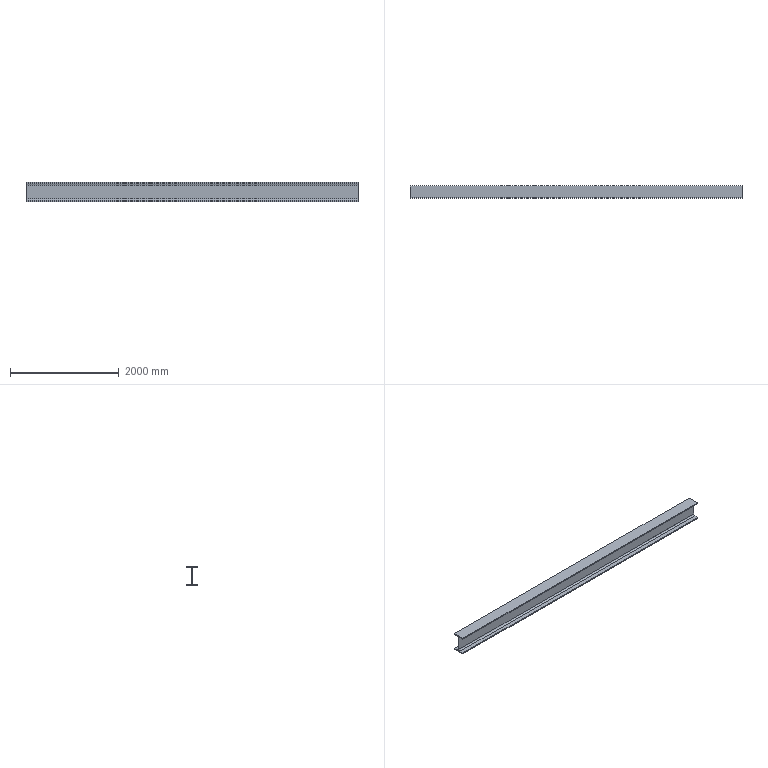Component | SolidWorks | OriginalColumn-2 | 1 solid | 18 faces | box 6100 x 220 x 350 mm | volume 80477247 mm3 | plane 14 | cylinder 4 | commonest cylinder face diameters 56 x4
build123d program:
from build123d import *

# Parameters (mm, degrees)
H_BEAM_HM600_300B_1_DEPTH = 6100


with BuildPart() as part:
    # Sketch1 → H-Beam HM600_300B_1 (new body)
    with BuildSketch(Plane.YZ):
        with BuildLine():
            Line((-110, -175), (-110, -155))
            Line((-110, -155), (-34, -155))
            ThreePointArc((-34, -155), (-14.201, -146.799), (-6, -127))
            Line((-6, -127), (-6, 127))
            ThreePointArc((-6, 127), (-14.201, 146.799), (-34, 155))
            Line((-34, 155), (-110, 155))
            Line((-110, 155), (-110, 175))
            Line((-110, 175), (110, 175))
            Line((110, 175), (110, 155))
            Line((110, 155), (34, 155))
            ThreePointArc((34, 155), (14.201, 146.799), (6, 127))
            Line((6, 127), (6, -127))
            ThreePointArc((6, -127), (14.201, -146.799), (34, -155))
            Line((34, -155), (110, -155))
            Line((110, -155), (110, -175))
            Line((110, -175), (-110, -175))
        make_face()
    extrude(amount=H_BEAM_HM600_300B_1_DEPTH)


solid = part.part

# Placed as in the assembly
solid = solid.moved(Location((-1730.074, -5132.346, -322.679), (0, 0, 0)))
STEP:
#1=COLOUR_RGB('',0.7922,0.8196,0.9333);
#2=FILL_AREA_STYLE_COLOUR('',#1);
#3=FILL_AREA_STYLE('',(#2));
#4=SURFACE_STYLE_FILL_AREA(#3);
#5=SURFACE_SIDE_STYLE('',(#4));
#6=SURFACE_STYLE_USAGE(.BOTH.,#5);
#7=PRESENTATION_STYLE_ASSIGNMENT((#6));
#8=CARTESIAN_POINT('',(-68.113,-206.392,-19.594));
#9=VERTEX_POINT('',#8);
#10=CARTESIAN_POINT('',(-68.113,-197.73,-19.594));
#11=VERTEX_POINT('',#10);
#12=CARTESIAN_POINT('',(-68.113,-197.73,-19.594));
#13=DIRECTION('',(0.,1.,0.));
#14=VECTOR('',#13,39.37);
#15=LINE('',#12,#14);
#16=EDGE_CURVE('',#9,#11,#15,.T.);
#17=ORIENTED_EDGE('',*,*,#16,.T.);
#18=CARTESIAN_POINT('',(172.044,-197.73,-19.594));
#19=VERTEX_POINT('',#18);
#20=CARTESIAN_POINT('',(172.044,-197.73,-19.594));
#21=DIRECTION('',(-1.,0.,0.));
#22=VECTOR('',#21,39.37);
#23=LINE('',#20,#22);
#24=EDGE_CURVE('',#19,#11,#23,.T.);
#25=ORIENTED_EDGE('',*,*,#24,.F.);
#26=CARTESIAN_POINT('',(172.044,-206.392,-19.594));
#27=VERTEX_POINT('',#26);
#28=CARTESIAN_POINT('',(172.044,-197.73,-19.594));
#29=DIRECTION('',(0.,1.,0.));
#30=VECTOR('',#29,39.37);
#31=LINE('',#28,#30);
#32=EDGE_CURVE('',#27,#19,#31,.T.);
#33=ORIENTED_EDGE('',*,*,#32,.F.);
#34=CARTESIAN_POINT('',(172.044,-206.392,-19.594));
#35=DIRECTION('',(-1.,0.,0.));
#36=VECTOR('',#35,39.37);
#37=LINE('',#34,#36);
#38=EDGE_CURVE('',#27,#9,#37,.T.);
#39=ORIENTED_EDGE('',*,*,#38,.T.);
#40=EDGE_LOOP('',(#17,#25,#33,#39));
#41=FACE_OUTER_BOUND('',#40,.T.);
#42=CARTESIAN_POINT('',(172.044,-197.73,-19.594));
#43=DIRECTION('',(0.,0.,1.));
#44=DIRECTION('',(1.,0.,0.));
#45=AXIS2_PLACEMENT_3D('',#42,#43,#44);
#46=PLANE('',#45);
#47=ADVANCED_FACE('',(#41),#46,.F.);
#48=CARTESIAN_POINT('',(-68.113,-197.73,-18.806));
#49=VERTEX_POINT('',#48);
#50=CARTESIAN_POINT('',(-68.113,-197.73,-18.806));
#51=DIRECTION('',(0.,0.,1.));
#52=VECTOR('',#51,39.37);
#53=LINE('',#50,#52);
#54=EDGE_CURVE('',#11,#49,#53,.T.);
#55=ORIENTED_EDGE('',*,*,#54,.T.);
#56=CARTESIAN_POINT('',(172.044,-197.73,-18.806));
#57=VERTEX_POINT('',#56);
#58=CARTESIAN_POINT('',(172.044,-197.73,-18.806));
#59=DIRECTION('',(-1.,0.,0.));
#60=VECTOR('',#59,39.37);
#61=LINE('',#58,#60);
#62=EDGE_CURVE('',#57,#49,#61,.T.);
#63=ORIENTED_EDGE('',*,*,#62,.F.);
#64=CARTESIAN_POINT('',(172.044,-197.73,-18.806));
#65=DIRECTION('',(0.,0.,1.));
#66=VECTOR('',#65,39.37);
#67=LINE('',#64,#66);
#68=EDGE_CURVE('',#19,#57,#67,.T.);
#69=ORIENTED_EDGE('',*,*,#68,.F.);
#70=ORIENTED_EDGE('',*,*,#24,.T.);
#71=EDGE_LOOP('',(#55,#63,#69,#70));
#72=FACE_OUTER_BOUND('',#71,.T.);
#73=CARTESIAN_POINT('',(172.044,-197.73,-18.806));
#74=DIRECTION('',(0.,-1.,0.));
#75=DIRECTION('',(0.,0.,-1.));
#76=AXIS2_PLACEMENT_3D('',#73,#74,#75);
#77=PLANE('',#76);
#78=ADVANCED_FACE('',(#72),#77,.F.);
#79=CARTESIAN_POINT('',(-68.113,-200.722,-18.806));
#80=VERTEX_POINT('',#79);
#81=CARTESIAN_POINT('',(-68.113,-197.73,-18.806));
#82=DIRECTION('',(0.,-1.,-0.));
#83=VECTOR('',#82,39.37);
#84=LINE('',#81,#83);
#85=EDGE_CURVE('',#49,#80,#84,.T.);
#86=ORIENTED_EDGE('',*,*,#85,.T.);
#87=CARTESIAN_POINT('',(172.044,-200.722,-18.806));
#88=VERTEX_POINT('',#87);
#89=CARTESIAN_POINT('',(172.044,-200.722,-18.806));
#90=DIRECTION('',(-1.,0.,0.));
#91=VECTOR('',#90,39.37);
#92=LINE('',#89,#91);
#93=EDGE_CURVE('',#88,#80,#92,.T.);
#94=ORIENTED_EDGE('',*,*,#93,.F.);
#95=CARTESIAN_POINT('',(172.044,-197.73,-18.806));
#96=DIRECTION('',(0.,-1.,-0.));
#97=VECTOR('',#96,39.37);
#98=LINE('',#95,#97);
#99=EDGE_CURVE('',#57,#88,#98,.T.);
#100=ORIENTED_EDGE('',*,*,#99,.F.);
#101=ORIENTED_EDGE('',*,*,#62,.T.);
#102=EDGE_LOOP('',(#86,#94,#100,#101));
#103=FACE_OUTER_BOUND('',#102,.T.);
#104=CARTESIAN_POINT('',(172.044,-197.73,-18.806));
#105=DIRECTION('',(0.,0.,-1.));
#106=DIRECTION('',(0.,1.,0.));
#107=AXIS2_PLACEMENT_3D('',#104,#105,#106);
#108=PLANE('',#107);
#109=ADVANCED_FACE('',(#103),#108,.F.);
#110=CARTESIAN_POINT('',(-68.113,-201.825,-17.704));
#111=VERTEX_POINT('',#110);
#112=CARTESIAN_POINT('',(-68.113,-200.722,-17.704));
#113=DIRECTION('',(-1.,0.,0.));
#114=DIRECTION('',(0.,0.,1.));
#115=AXIS2_PLACEMENT_3D('',#112,#113,#114);
#116=CIRCLE('',#115,1.102);
#117=EDGE_CURVE('',#80,#111,#116,.T.);
#118=ORIENTED_EDGE('',*,*,#117,.T.);
#119=CARTESIAN_POINT('',(172.044,-201.825,-17.704));
#120=VERTEX_POINT('',#119);
#121=CARTESIAN_POINT('',(172.044,-201.825,-17.704));
#122=DIRECTION('',(-1.,0.,0.));
#123=VECTOR('',#122,39.37);
#124=LINE('',#121,#123);
#125=EDGE_CURVE('',#120,#111,#124,.T.);
#126=ORIENTED_EDGE('',*,*,#125,.F.);
#127=CARTESIAN_POINT('',(172.044,-200.722,-17.704));
#128=DIRECTION('',(-1.,0.,0.));
#129=DIRECTION('',(0.,0.,1.));
#130=AXIS2_PLACEMENT_3D('',#127,#128,#129);
#131=CIRCLE('',#130,1.102);
#132=EDGE_CURVE('',#88,#120,#131,.T.);
#133=ORIENTED_EDGE('',*,*,#132,.F.);
#134=ORIENTED_EDGE('',*,*,#93,.T.);
#135=EDGE_LOOP('',(#118,#126,#133,#134));
#136=FACE_OUTER_BOUND('',#135,.T.);
#137=CARTESIAN_POINT('',(172.044,-200.722,-17.704));
#138=DIRECTION('',(-1.,0.,0.));
#139=DIRECTION('',(0.,0.,1.));
#140=AXIS2_PLACEMENT_3D('',#137,#138,#139);
#141=CYLINDRICAL_SURFACE('',#140,1.102);
#142=ADVANCED_FACE('',(#136),#141,.F.);
#143=CARTESIAN_POINT('',(-68.113,-201.825,-7.704));
#144=VERTEX_POINT('',#143);
#145=CARTESIAN_POINT('',(-68.113,-201.825,-7.704));
#146=DIRECTION('',(0.,-0.,1.));
#147=VECTOR('',#146,39.37);
#148=LINE('',#145,#147);
#149=EDGE_CURVE('',#111,#144,#148,.T.);
#150=ORIENTED_EDGE('',*,*,#149,.T.);
#151=CARTESIAN_POINT('',(172.044,-201.825,-7.704));
#152=VERTEX_POINT('',#151);
#153=CARTESIAN_POINT('',(172.044,-201.825,-7.704));
#154=DIRECTION('',(-1.,0.,0.));
#155=VECTOR('',#154,39.37);
#156=LINE('',#153,#155);
#157=EDGE_CURVE('',#152,#144,#156,.T.);
#158=ORIENTED_EDGE('',*,*,#157,.F.);
#159=CARTESIAN_POINT('',(172.044,-201.825,-7.704));
#160=DIRECTION('',(0.,-0.,1.));
#161=VECTOR('',#160,39.37);
#162=LINE('',#159,#161);
#163=EDGE_CURVE('',#120,#152,#162,.T.);
#164=ORIENTED_EDGE('',*,*,#163,.F.);
#165=ORIENTED_EDGE('',*,*,#125,.T.);
#166=EDGE_LOOP('',(#150,#158,#164,#165));
#167=FACE_OUTER_BOUND('',#166,.T.);
#168=CARTESIAN_POINT('',(172.044,-201.825,-7.704));
#169=DIRECTION('',(0.,-1.,-0.));
#170=DIRECTION('',(0.,0.,-1.));
#171=AXIS2_PLACEMENT_3D('',#168,#169,#170);
#172=PLANE('',#171);
#173=ADVANCED_FACE('',(#167),#172,.F.);
#174=CARTESIAN_POINT('',(-68.113,-200.722,-6.602));
#175=VERTEX_POINT('',#174);
#176=CARTESIAN_POINT('',(-68.113,-200.722,-7.704));
#177=DIRECTION('',(-1.,0.,0.));
#178=DIRECTION('',(0.,0.,1.));
#179=AXIS2_PLACEMENT_3D('',#176,#177,#178);
#180=CIRCLE('',#179,1.102);
#181=EDGE_CURVE('',#144,#175,#180,.T.);
#182=ORIENTED_EDGE('',*,*,#181,.T.);
#183=CARTESIAN_POINT('',(172.044,-200.722,-6.602));
#184=VERTEX_POINT('',#183);
#185=CARTESIAN_POINT('',(172.044,-200.722,-6.602));
#186=DIRECTION('',(-1.,0.,0.));
#187=VECTOR('',#186,39.37);
#188=LINE('',#185,#187);
#189=EDGE_CURVE('',#184,#175,#188,.T.);
#190=ORIENTED_EDGE('',*,*,#189,.F.);
#191=CARTESIAN_POINT('',(172.044,-200.722,-7.704));
#192=DIRECTION('',(-1.,0.,0.));
#193=DIRECTION('',(0.,0.,1.));
#194=AXIS2_PLACEMENT_3D('',#191,#192,#193);
#195=CIRCLE('',#194,1.102);
#196=EDGE_CURVE('',#152,#184,#195,.T.);
#197=ORIENTED_EDGE('',*,*,#196,.F.);
#198=ORIENTED_EDGE('',*,*,#157,.T.);
#199=EDGE_LOOP('',(#182,#190,#197,#198));
#200=FACE_OUTER_BOUND('',#199,.T.);
#201=CARTESIAN_POINT('',(172.044,-200.722,-7.704));
#202=DIRECTION('',(-1.,0.,0.));
#203=DIRECTION('',(0.,0.,1.));
#204=AXIS2_PLACEMENT_3D('',#201,#202,#203);
#205=CYLINDRICAL_SURFACE('',#204,1.102);
#206=ADVANCED_FACE('',(#200),#205,.F.);
#207=CARTESIAN_POINT('',(-68.113,-197.73,-6.602));
#208=VERTEX_POINT('',#207);
#209=CARTESIAN_POINT('',(-68.113,-200.722,-6.602));
#210=DIRECTION('',(0.,1.,-0.));
#211=VECTOR('',#210,39.37);
#212=LINE('',#209,#211);
#213=EDGE_CURVE('',#175,#208,#212,.T.);
#214=ORIENTED_EDGE('',*,*,#213,.T.);
#215=CARTESIAN_POINT('',(172.044,-197.73,-6.602));
#216=VERTEX_POINT('',#215);
#217=CARTESIAN_POINT('',(172.044,-197.73,-6.602));
#218=DIRECTION('',(-1.,0.,0.));
#219=VECTOR('',#218,39.37);
#220=LINE('',#217,#219);
#221=EDGE_CURVE('',#216,#208,#220,.T.);
#222=ORIENTED_EDGE('',*,*,#221,.F.);
#223=CARTESIAN_POINT('',(172.044,-200.722,-6.602));
#224=DIRECTION('',(0.,1.,-0.));
#225=VECTOR('',#224,39.37);
#226=LINE('',#223,#225);
#227=EDGE_CURVE('',#184,#216,#226,.T.);
#228=ORIENTED_EDGE('',*,*,#227,.F.);
#229=ORIENTED_EDGE('',*,*,#189,.T.);
#230=EDGE_LOOP('',(#214,#222,#228,#229));
#231=FACE_OUTER_BOUND('',#230,.T.);
#232=CARTESIAN_POINT('',(172.044,-200.722,-6.602));
#233=DIRECTION('',(0.,0.,1.));
#234=DIRECTION('',(0.,-1.,0.));
#235=AXIS2_PLACEMENT_3D('',#232,#233,#234);
#236=PLANE('',#235);
#237=ADVANCED_FACE('',(#231),#236,.F.);
#238=CARTESIAN_POINT('',(-68.113,-197.73,-5.814));
#239=VERTEX_POINT('',#238);
#240=CARTESIAN_POINT('',(-68.113,-197.73,-5.814));
#241=DIRECTION('',(0.,0.,1.));
#242=VECTOR('',#241,39.37);
#243=LINE('',#240,#242);
#244=EDGE_CURVE('',#208,#239,#243,.T.);
#245=ORIENTED_EDGE('',*,*,#244,.T.);
#246=CARTESIAN_POINT('',(172.044,-197.73,-5.814));
#247=VERTEX_POINT('',#246);
#248=CARTESIAN_POINT('',(172.044,-197.73,-5.814));
#249=DIRECTION('',(-1.,0.,0.));
#250=VECTOR('',#249,39.37);
#251=LINE('',#248,#250);
#252=EDGE_CURVE('',#247,#239,#251,.T.);
#253=ORIENTED_EDGE('',*,*,#252,.F.);
#254=CARTESIAN_POINT('',(172.044,-197.73,-5.814));
#255=DIRECTION('',(0.,0.,1.));
#256=VECTOR('',#255,39.37);
#257=LINE('',#254,#256);
#258=EDGE_CURVE('',#216,#247,#257,.T.);
#259=ORIENTED_EDGE('',*,*,#258,.F.);
#260=ORIENTED_EDGE('',*,*,#221,.T.);
#261=EDGE_LOOP('',(#245,#253,#259,#260));
#262=FACE_OUTER_BOUND('',#261,.T.);
#263=CARTESIAN_POINT('',(172.044,-197.73,-5.814));
#264=DIRECTION('',(0.,-1.,0.));
#265=DIRECTION('',(0.,0.,-1.));
#266=AXIS2_PLACEMENT_3D('',#263,#264,#265);
#267=PLANE('',#266);
#268=ADVANCED_FACE('',(#262),#267,.F.);
#269=CARTESIAN_POINT('',(-68.113,-206.392,-5.814));
#270=VERTEX_POINT('',#269);
#271=CARTESIAN_POINT('',(-68.113,-206.392,-5.814));
#272=DIRECTION('',(0.,-1.,0.));
#273=VECTOR('',#272,39.37);
#274=LINE('',#271,#273);
#275=EDGE_CURVE('',#239,#270,#274,.T.);
#276=ORIENTED_EDGE('',*,*,#275,.T.);
#277=CARTESIAN_POINT('',(172.044,-206.392,-5.814));
#278=VERTEX_POINT('',#277);
#279=CARTESIAN_POINT('',(172.044,-206.392,-5.814));
#280=DIRECTION('',(-1.,0.,0.));
#281=VECTOR('',#280,39.37);
#282=LINE('',#279,#281);
#283=EDGE_CURVE('',#278,#270,#282,.T.);
#284=ORIENTED_EDGE('',*,*,#283,.F.);
#285=CARTESIAN_POINT('',(172.044,-206.392,-5.814));
#286=DIRECTION('',(0.,-1.,0.));
#287=VECTOR('',#286,39.37);
#288=LINE('',#285,#287);
#289=EDGE_CURVE('',#247,#278,#288,.T.);
#290=ORIENTED_EDGE('',*,*,#289,.F.);
#291=ORIENTED_EDGE('',*,*,#252,.T.);
#292=EDGE_LOOP('',(#276,#284,#290,#291));
#293=FACE_OUTER_BOUND('',#292,.T.);
#294=CARTESIAN_POINT('',(172.044,-206.392,-5.814));
#295=DIRECTION('',(0.,0.,-1.));
#296=DIRECTION('',(-1.,0.,0.));
#297=AXIS2_PLACEMENT_3D('',#294,#295,#296);
#298=PLANE('',#297);
#299=ADVANCED_FACE('',(#293),#298,.F.);
#300=CARTESIAN_POINT('',(-68.113,-206.392,-6.602));
#301=VERTEX_POINT('',#300);
#302=CARTESIAN_POINT('',(-68.113,-206.392,-6.602));
#303=DIRECTION('',(0.,0.,-1.));
#304=VECTOR('',#303,39.37);
#305=LINE('',#302,#304);
#306=EDGE_CURVE('',#270,#301,#305,.T.);
#307=ORIENTED_EDGE('',*,*,#306,.T.);
#308=CARTESIAN_POINT('',(172.044,-206.392,-6.602));
#309=VERTEX_POINT('',#308);
#310=CARTESIAN_POINT('',(172.044,-206.392,-6.602));
#311=DIRECTION('',(-1.,0.,0.));
#312=VECTOR('',#311,39.37);
#313=LINE('',#310,#312);
#314=EDGE_CURVE('',#309,#301,#313,.T.);
#315=ORIENTED_EDGE('',*,*,#314,.F.);
#316=CARTESIAN_POINT('',(172.044,-206.392,-6.602));
#317=DIRECTION('',(0.,0.,-1.));
#318=VECTOR('',#317,39.37);
#319=LINE('',#316,#318);
#320=EDGE_CURVE('',#278,#309,#319,.T.);
#321=ORIENTED_EDGE('',*,*,#320,.F.);
#322=ORIENTED_EDGE('',*,*,#283,.T.);
#323=EDGE_LOOP('',(#307,#315,#321,#322));
#324=FACE_OUTER_BOUND('',#323,.T.);
#325=CARTESIAN_POINT('',(172.044,-206.392,-6.602));
#326=DIRECTION('',(0.,1.,0.));
#327=DIRECTION('',(0.,0.,1.));
#328=AXIS2_PLACEMENT_3D('',#325,#326,#327);
#329=PLANE('',#328);
#330=ADVANCED_FACE('',(#324),#329,.F.);
#331=CARTESIAN_POINT('',(-68.113,-203.399,-6.602));
#332=VERTEX_POINT('',#331);
#333=CARTESIAN_POINT('',(-68.113,-206.392,-6.602));
#334=DIRECTION('',(0.,1.,0.));
#335=VECTOR('',#334,39.37);
#336=LINE('',#333,#335);
#337=EDGE_CURVE('',#301,#332,#336,.T.);
#338=ORIENTED_EDGE('',*,*,#337,.T.);
#339=CARTESIAN_POINT('',(172.044,-203.399,-6.602));
#340=VERTEX_POINT('',#339);
#341=CARTESIAN_POINT('',(172.044,-203.399,-6.602));
#342=DIRECTION('',(-1.,0.,0.));
#343=VECTOR('',#342,39.37);
#344=LINE('',#341,#343);
#345=EDGE_CURVE('',#340,#332,#344,.T.);
#346=ORIENTED_EDGE('',*,*,#345,.F.);
#347=CARTESIAN_POINT('',(172.044,-206.392,-6.602));
#348=DIRECTION('',(0.,1.,0.));
#349=VECTOR('',#348,39.37);
#350=LINE('',#347,#349);
#351=EDGE_CURVE('',#309,#340,#350,.T.);
#352=ORIENTED_EDGE('',*,*,#351,.F.);
#353=ORIENTED_EDGE('',*,*,#314,.T.);
#354=EDGE_LOOP('',(#338,#346,#352,#353));
#355=FACE_OUTER_BOUND('',#354,.T.);
#356=CARTESIAN_POINT('',(172.044,-206.392,-6.602));
#357=DIRECTION('',(0.,-0.,1.));
#358=DIRECTION('',(0.,-1.,-0.));
#359=AXIS2_PLACEMENT_3D('',#356,#357,#358);
#360=PLANE('',#359);
#361=ADVANCED_FACE('',(#355),#360,.F.);
#362=CARTESIAN_POINT('',(-68.113,-202.297,-7.704));
#363=VERTEX_POINT('',#362);
#364=CARTESIAN_POINT('',(-68.113,-203.399,-7.704));
#365=DIRECTION('',(-1.,0.,0.));
#366=DIRECTION('',(0.,0.,-1.));
#367=AXIS2_PLACEMENT_3D('',#364,#365,#366);
#368=CIRCLE('',#367,1.102);
#369=EDGE_CURVE('',#332,#363,#368,.T.);
#370=ORIENTED_EDGE('',*,*,#369,.T.);
#371=CARTESIAN_POINT('',(172.044,-202.297,-7.704));
#372=VERTEX_POINT('',#371);
#373=CARTESIAN_POINT('',(172.044,-202.297,-7.704));
#374=DIRECTION('',(-1.,0.,0.));
#375=VECTOR('',#374,39.37);
#376=LINE('',#373,#375);
#377=EDGE_CURVE('',#372,#363,#376,.T.);
#378=ORIENTED_EDGE('',*,*,#377,.F.);
#379=CARTESIAN_POINT('',(172.044,-203.399,-7.704));
#380=DIRECTION('',(-1.,0.,0.));
#381=DIRECTION('',(0.,0.,-1.));
#382=AXIS2_PLACEMENT_3D('',#379,#380,#381);
#383=CIRCLE('',#382,1.102);
#384=EDGE_CURVE('',#340,#372,#383,.T.);
#385=ORIENTED_EDGE('',*,*,#384,.F.);
#386=ORIENTED_EDGE('',*,*,#345,.T.);
#387=EDGE_LOOP('',(#370,#378,#385,#386));
#388=FACE_OUTER_BOUND('',#387,.T.);
#389=CARTESIAN_POINT('',(172.044,-203.399,-7.704));
#390=DIRECTION('',(-1.,0.,0.));
#391=DIRECTION('',(0.,0.,1.));
#392=AXIS2_PLACEMENT_3D('',#389,#390,#391);
#393=CYLINDRICAL_SURFACE('',#392,1.102);
#394=ADVANCED_FACE('',(#388),#393,.F.);
#395=CARTESIAN_POINT('',(-68.113,-202.297,-17.704));
#396=VERTEX_POINT('',#395);
#397=CARTESIAN_POINT('',(-68.113,-202.297,-17.704));
#398=DIRECTION('',(0.,0.,-1.));
#399=VECTOR('',#398,39.37);
#400=LINE('',#397,#399);
#401=EDGE_CURVE('',#363,#396,#400,.T.);
#402=ORIENTED_EDGE('',*,*,#401,.T.);
#403=CARTESIAN_POINT('',(172.044,-202.297,-17.704));
#404=VERTEX_POINT('',#403);
#405=CARTESIAN_POINT('',(172.044,-202.297,-17.704));
#406=DIRECTION('',(-1.,0.,0.));
#407=VECTOR('',#406,39.37);
#408=LINE('',#405,#407);
#409=EDGE_CURVE('',#404,#396,#408,.T.);
#410=ORIENTED_EDGE('',*,*,#409,.F.);
#411=CARTESIAN_POINT('',(172.044,-202.297,-17.704));
#412=DIRECTION('',(0.,0.,-1.));
#413=VECTOR('',#412,39.37);
#414=LINE('',#411,#413);
#415=EDGE_CURVE('',#372,#404,#414,.T.);
#416=ORIENTED_EDGE('',*,*,#415,.F.);
#417=ORIENTED_EDGE('',*,*,#377,.T.);
#418=EDGE_LOOP('',(#402,#410,#416,#417));
#419=FACE_OUTER_BOUND('',#418,.T.);
#420=CARTESIAN_POINT('',(172.044,-202.297,-17.704));
#421=DIRECTION('',(0.,1.,0.));
#422=DIRECTION('',(0.,-0.,1.));
#423=AXIS2_PLACEMENT_3D('',#420,#421,#422);
#424=PLANE('',#423);
#425=ADVANCED_FACE('',(#419),#424,.F.);
#426=CARTESIAN_POINT('',(-68.113,-203.399,-18.806));
#427=VERTEX_POINT('',#426);
#428=CARTESIAN_POINT('',(-68.113,-203.399,-17.704));
#429=DIRECTION('',(-1.,0.,0.));
#430=DIRECTION('',(0.,0.,-1.));
#431=AXIS2_PLACEMENT_3D('',#428,#429,#430);
#432=CIRCLE('',#431,1.102);
#433=EDGE_CURVE('',#396,#427,#432,.T.);
#434=ORIENTED_EDGE('',*,*,#433,.T.);
#435=CARTESIAN_POINT('',(172.044,-203.399,-18.806));
#436=VERTEX_POINT('',#435);
#437=CARTESIAN_POINT('',(172.044,-203.399,-18.806));
#438=DIRECTION('',(-1.,0.,0.));
#439=VECTOR('',#438,39.37);
#440=LINE('',#437,#439);
#441=EDGE_CURVE('',#436,#427,#440,.T.);
#442=ORIENTED_EDGE('',*,*,#441,.F.);
#443=CARTESIAN_POINT('',(172.044,-203.399,-17.704));
#444=DIRECTION('',(-1.,0.,0.));
#445=DIRECTION('',(0.,0.,-1.));
#446=AXIS2_PLACEMENT_3D('',#443,#444,#445);
#447=CIRCLE('',#446,1.102);
#448=EDGE_CURVE('',#404,#436,#447,.T.);
#449=ORIENTED_EDGE('',*,*,#448,.F.);
#450=ORIENTED_EDGE('',*,*,#409,.T.);
#451=EDGE_LOOP('',(#434,#442,#449,#450));
#452=FACE_OUTER_BOUND('',#451,.T.);
#453=CARTESIAN_POINT('',(172.044,-203.399,-17.704));
#454=DIRECTION('',(-1.,0.,0.));
#455=DIRECTION('',(0.,0.,1.));
#456=AXIS2_PLACEMENT_3D('',#453,#454,#455);
#457=CYLINDRICAL_SURFACE('',#456,1.102);
#458=ADVANCED_FACE('',(#452),#457,.F.);
#459=CARTESIAN_POINT('',(-68.113,-206.392,-18.806));
#460=VERTEX_POINT('',#459);
#461=CARTESIAN_POINT('',(-68.113,-203.399,-18.806));
#462=DIRECTION('',(0.,-1.,0.));
#463=VECTOR('',#462,39.37);
#464=LINE('',#461,#463);
#465=EDGE_CURVE('',#427,#460,#464,.T.);
#466=ORIENTED_EDGE('',*,*,#465,.T.);
#467=CARTESIAN_POINT('',(172.044,-206.392,-18.806));
#468=VERTEX_POINT('',#467);
#469=CARTESIAN_POINT('',(172.044,-206.392,-18.806));
#470=DIRECTION('',(-1.,0.,0.));
#471=VECTOR('',#470,39.37);
#472=LINE('',#469,#471);
#473=EDGE_CURVE('',#468,#460,#472,.T.);
#474=ORIENTED_EDGE('',*,*,#473,.F.);
#475=CARTESIAN_POINT('',(172.044,-203.399,-18.806));
#476=DIRECTION('',(0.,-1.,0.));
#477=VECTOR('',#476,39.37);
#478=LINE('',#475,#477);
#479=EDGE_CURVE('',#436,#468,#478,.T.);
#480=ORIENTED_EDGE('',*,*,#479,.F.);
#481=ORIENTED_EDGE('',*,*,#441,.T.);
#482=EDGE_LOOP('',(#466,#474,#480,#481));
#483=FACE_OUTER_BOUND('',#482,.T.);
#484=CARTESIAN_POINT('',(172.044,-203.399,-18.806));
#485=DIRECTION('',(0.,-0.,-1.));
#486=DIRECTION('',(0.,1.,-0.));
#487=AXIS2_PLACEMENT_3D('',#484,#485,#486);
#488=PLANE('',#487);
#489=ADVANCED_FACE('',(#483),#488,.F.);
#490=CARTESIAN_POINT('',(-68.113,-206.392,-19.594));
#491=DIRECTION('',(0.,-0.,-1.));
#492=VECTOR('',#491,39.37);
#493=LINE('',#490,#492);
#494=EDGE_CURVE('',#460,#9,#493,.T.);
#495=ORIENTED_EDGE('',*,*,#494,.T.);
#496=ORIENTED_EDGE('',*,*,#38,.F.);
#497=CARTESIAN_POINT('',(172.044,-206.392,-19.594));
#498=DIRECTION('',(0.,-0.,-1.));
#499=VECTOR('',#498,39.37);
#500=LINE('',#497,#499);
#501=EDGE_CURVE('',#468,#27,#500,.T.);
#502=ORIENTED_EDGE('',*,*,#501,.F.);
#503=ORIENTED_EDGE('',*,*,#473,.T.);
#504=EDGE_LOOP('',(#495,#496,#502,#503));
#505=FACE_OUTER_BOUND('',#504,.T.);
#506=CARTESIAN_POINT('',(172.044,-206.392,-19.594));
#507=DIRECTION('',(0.,1.,-0.));
#508=DIRECTION('',(0.,0.,1.));
#509=AXIS2_PLACEMENT_3D('',#506,#507,#508);
#510=PLANE('',#509);
#511=ADVANCED_FACE('',(#505),#510,.F.);
#512=ORIENTED_EDGE('',*,*,#32,.T.);
#513=ORIENTED_EDGE('',*,*,#68,.T.);
#514=ORIENTED_EDGE('',*,*,#99,.T.);
#515=ORIENTED_EDGE('',*,*,#132,.T.);
#516=ORIENTED_EDGE('',*,*,#163,.T.);
#517=ORIENTED_EDGE('',*,*,#196,.T.);
#518=ORIENTED_EDGE('',*,*,#227,.T.);
#519=ORIENTED_EDGE('',*,*,#258,.T.);
#520=ORIENTED_EDGE('',*,*,#289,.T.);
#521=ORIENTED_EDGE('',*,*,#320,.T.);
#522=ORIENTED_EDGE('',*,*,#351,.T.);
#523=ORIENTED_EDGE('',*,*,#384,.T.);
#524=ORIENTED_EDGE('',*,*,#415,.T.);
#525=ORIENTED_EDGE('',*,*,#448,.T.);
#526=ORIENTED_EDGE('',*,*,#479,.T.);
#527=ORIENTED_EDGE('',*,*,#501,.T.);
#528=EDGE_LOOP('',(#512,#513,#514,#515,#516,#517,#518,#519,#520,#521,#522,#523,#524,#525,#526,#527));
#529=FACE_OUTER_BOUND('',#528,.T.);
#530=CARTESIAN_POINT('',(172.044,-203.399,-17.704));
#531=DIRECTION('',(1.,0.,0.));
#532=DIRECTION('',(0.,0.,-1.));
#533=AXIS2_PLACEMENT_3D('',#530,#531,#532);
#534=PLANE('',#533);
#535=ADVANCED_FACE('',(#529),#534,.T.);
#536=ORIENTED_EDGE('',*,*,#16,.F.);
#537=ORIENTED_EDGE('',*,*,#494,.F.);
#538=ORIENTED_EDGE('',*,*,#465,.F.);
#539=ORIENTED_EDGE('',*,*,#433,.F.);
#540=ORIENTED_EDGE('',*,*,#401,.F.);
#541=ORIENTED_EDGE('',*,*,#369,.F.);
#542=ORIENTED_EDGE('',*,*,#337,.F.);
#543=ORIENTED_EDGE('',*,*,#306,.F.);
#544=ORIENTED_EDGE('',*,*,#275,.F.);
#545=ORIENTED_EDGE('',*,*,#244,.F.);
#546=ORIENTED_EDGE('',*,*,#213,.F.);
#547=ORIENTED_EDGE('',*,*,#181,.F.);
#548=ORIENTED_EDGE('',*,*,#149,.F.);
#549=ORIENTED_EDGE('',*,*,#117,.F.);
#550=ORIENTED_EDGE('',*,*,#85,.F.);
#551=ORIENTED_EDGE('',*,*,#54,.F.);
#552=EDGE_LOOP('',(#536,#537,#538,#539,#540,#541,#542,#543,#544,#545,#546,#547,#548,#549,#550,#551));
#553=FACE_OUTER_BOUND('',#552,.T.);
#554=CARTESIAN_POINT('',(-68.113,-203.399,-17.704));
#555=DIRECTION('',(1.,0.,0.));
#556=DIRECTION('',(0.,0.,-1.));
#557=AXIS2_PLACEMENT_3D('',#554,#555,#556);
#558=PLANE('',#557);
#559=ADVANCED_FACE('',(#553),#558,.F.);
#560=CLOSED_SHELL('',(#47,#78,#109,#142,#173,#206,#237,#268,#299,#330,#361,#394,#425,#458,#489,#511,#535,#559));
#561=MANIFOLD_SOLID_BREP('',#560);
#562=STYLED_ITEM('',(#7),#561);
#563=(LENGTH_UNIT()NAMED_UNIT(*)SI_UNIT($,.METRE.));
#564=LENGTH_MEASURE_WITH_UNIT(LENGTH_MEASURE(0.0254),#563);
#565=DIMENSIONAL_EXPONENTS(1.,0.,0.,0.,0.,0.,0.);
#566=(CONVERSION_BASED_UNIT('',#564)LENGTH_UNIT()NAMED_UNIT(#565));
#567=UNCERTAINTY_MEASURE_WITH_UNIT(LENGTH_MEASURE(0.00001),#566,'','');
#568=(NAMED_UNIT(*)PLANE_ANGLE_UNIT()SI_UNIT($,.RADIAN.));
#569=(NAMED_UNIT(*)SI_UNIT($,.STERADIAN.)SOLID_ANGLE_UNIT());
#570=(GEOMETRIC_REPRESENTATION_CONTEXT(3)GLOBAL_UNCERTAINTY_ASSIGNED_CONTEXT((#567))GLOBAL_UNIT_ASSIGNED_CONTEXT((#566,#568,#569))REPRESENTATION_CONTEXT('',''));
#571=MECHANICAL_DESIGN_GEOMETRIC_PRESENTATION_REPRESENTATION('',(#562),#570);
#572=PRESENTATION_LAYER_ASSIGNMENT('','',(#562));
#573=CARTESIAN_POINT('',(0.,0.,0.));
#574=DIRECTION('',(0.,0.,1.));
#575=DIRECTION('',(1.,0.,0.));
#576=AXIS2_PLACEMENT_3D('',#573,#574,#575);
#577=(LENGTH_UNIT()NAMED_UNIT(*)SI_UNIT($,.METRE.));
#578=LENGTH_MEASURE_WITH_UNIT(LENGTH_MEASURE(0.0254),#577);
#579=DIMENSIONAL_EXPONENTS(1.,0.,0.,0.,0.,0.,0.);
#580=(CONVERSION_BASED_UNIT('',#578)LENGTH_UNIT()NAMED_UNIT(#579));
#581=UNCERTAINTY_MEASURE_WITH_UNIT(LENGTH_MEASURE(0.00001),#580,'','');
#582=(NAMED_UNIT(*)PLANE_ANGLE_UNIT()SI_UNIT($,.RADIAN.));
#583=(NAMED_UNIT(*)SI_UNIT($,.STERADIAN.)SOLID_ANGLE_UNIT());
#584=(GEOMETRIC_REPRESENTATION_CONTEXT(3)GLOBAL_UNCERTAINTY_ASSIGNED_CONTEXT((#581))GLOBAL_UNIT_ASSIGNED_CONTEXT((#580,#582,#583))REPRESENTATION_CONTEXT('',''));
#585=ADVANCED_BREP_SHAPE_REPRESENTATION('',(#561,#576),#584);